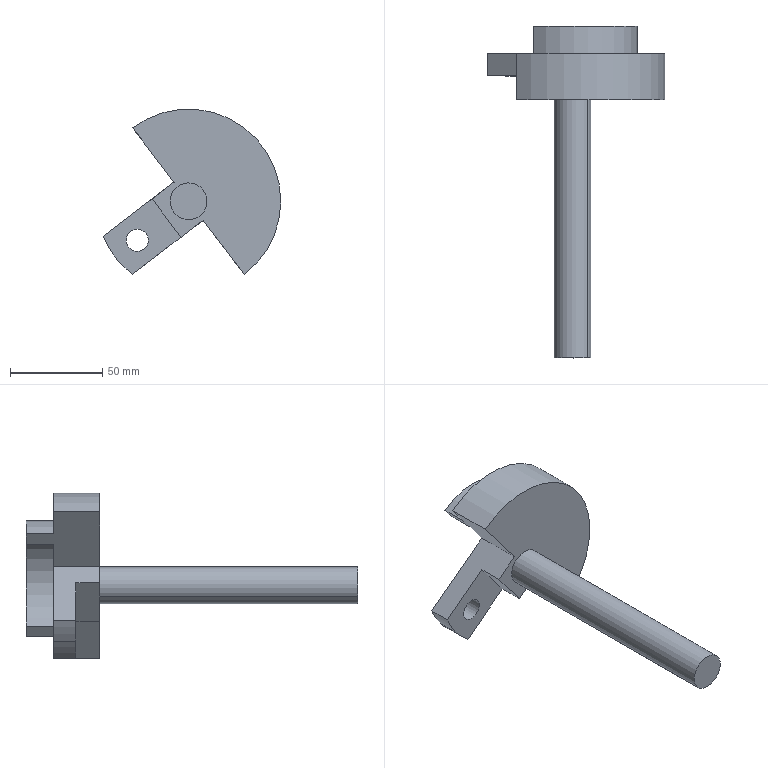Component | SolidWorks | RearRoller-4 | 1 solid | 20 faces | box 96.28 x 180 x 89.77 mm | volume 171683 mm3 | plane 11 | cylinder 9 | commonest cylinder face diameters 100 x3 12 x2 20 x2 56 x1 70 x1
build123d program:
from build123d import *

# Parameters (mm, degrees)
SKETCH2_W      = 83.89
SKETCH2_H      = 46.873
EXTRUDE2_DEPTH = 15
SKETCH3_W      = 56.676
SKETCH3_H      = 55.605
EXTRUDE3_DEPTH = 180.513
SKETCH4_R      = 6
EXTRUDE4_DEPTH = 180.513
SKETCH5_W      = 35
SKETCH5_H      = 13
EXTRUDE5_DEPTH = 148.923


with BuildPart() as part:
    # Sketch1 → Revolve1 (revolve)
    with BuildSketch(Plane.XY, mode=Mode.PRIVATE) as revolve1_sk:
        Polygon((0, 109.146), (28, 109.146), (28, 124.146), (35, 124.146), (35, 109.146), (50, 109.146), (50, 84.146), (10, 84.146), (10, -55.854), (0, -55.854), align=None)
    revolve(revolve1_sk.sketch.rotate(Axis((0, 0, 0), (0, 1, 0)), 90), axis=Axis((0, 0, 0), (0, 1, 0)))

    # Sketch2 → Extrude2 (cut)
    with BuildSketch(Plane(origin=(0, 124.146, 0), x_dir=(1, 0, 0), z_dir=(0, 1, 0))):
        with Locations((-6.945, 23.437)):
            Rectangle(SKETCH2_W, SKETCH2_H)
    extrude(amount=-EXTRUDE2_DEPTH, mode=Mode.SUBTRACT)

    # Sketch3 → Extrude3 (cut, through all)
    with BuildSketch(Plane(origin=(0, 109.146, 0), x_dir=(1, 0, 0), z_dir=(0, 1, 0))):
        with Locations((-41.338, 27.803)):
            Rectangle(SKETCH3_W, SKETCH3_H)
        with Locations((41.338, 27.803)):
            Rectangle(SKETCH3_W, SKETCH3_H)
    extrude(amount=-EXTRUDE3_DEPTH, mode=Mode.SUBTRACT)

    # Sketch4 → Extrude4 (cut, through all)
    with BuildSketch(Plane(origin=(0, 109.146, 0), x_dir=(1, 0, 0), z_dir=(0, 1, 0))):
        with Locations(Location((0, 35, 0), (0, 0, 270))):
            Circle(SKETCH4_R)
    extrude(amount=-EXTRUDE4_DEPTH, mode=Mode.SUBTRACT)

    # Sketch5 → Extrude5 (cut, through all)
    with BuildSketch(Plane(origin=(13, 0, 0), x_dir=(0, 0, -1), z_dir=(1, 0, 0))):
        with Locations((32.5, 90.646)):
            Rectangle(SKETCH5_W, SKETCH5_H)
    extrude(amount=-EXTRUDE5_DEPTH, mode=Mode.SUBTRACT)


solid = part.part

# Placed as in the assembly
solid = solid.moved(Location((-214.784, 404.838, -155), (0, 52.688, 0)))
STEP:
#1=COLOUR_RGB('',0.7922,0.8196,0.9333);
#2=FILL_AREA_STYLE_COLOUR('',#1);
#3=FILL_AREA_STYLE('',(#2));
#4=SURFACE_STYLE_FILL_AREA(#3);
#5=SURFACE_SIDE_STYLE('',(#4));
#6=SURFACE_STYLE_USAGE(.BOTH.,#5);
#7=PRESENTATION_STYLE_ASSIGNMENT((#6));
#8=CARTESIAN_POINT('',(-9.364,19.763,-6.794));
#9=VERTEX_POINT('',#8);
#10=CARTESIAN_POINT('',(-9.74,19.763,-7.081));
#11=VERTEX_POINT('',#10);
#12=CARTESIAN_POINT('',(-9.552,19.763,-6.938));
#13=DIRECTION('',(0.,-1.,-0.));
#14=DIRECTION('',(0.7953,0.,0.6062));
#15=AXIS2_PLACEMENT_3D('',#12,#13,#14);
#16=CIRCLE('',#15,0.2362);
#17=EDGE_CURVE('',#9,#11,#16,.T.);
#18=ORIENTED_EDGE('',*,*,#17,.T.);
#19=CARTESIAN_POINT('',(-9.74,20.236,-7.081));
#20=VERTEX_POINT('',#19);
#21=CARTESIAN_POINT('',(-9.74,13.74,-7.081));
#22=DIRECTION('',(-0.,1.,0.));
#23=VECTOR('',#22,39.37);
#24=LINE('',#21,#23);
#25=EDGE_CURVE('',#11,#20,#24,.T.);
#26=ORIENTED_EDGE('',*,*,#25,.T.);
#27=CARTESIAN_POINT('',(-9.364,20.236,-6.794));
#28=VERTEX_POINT('',#27);
#29=CARTESIAN_POINT('',(-9.552,20.236,-6.938));
#30=DIRECTION('',(-0.,1.,0.));
#31=DIRECTION('',(0.7953,0.,0.6062));
#32=AXIS2_PLACEMENT_3D('',#29,#30,#31);
#33=CIRCLE('',#32,0.2362);
#34=EDGE_CURVE('',#20,#28,#33,.T.);
#35=ORIENTED_EDGE('',*,*,#34,.T.);
#36=CARTESIAN_POINT('',(-9.364,13.74,-6.794));
#37=DIRECTION('',(-0.,1.,0.));
#38=VECTOR('',#37,39.37);
#39=LINE('',#36,#38);
#40=EDGE_CURVE('',#9,#28,#39,.T.);
#41=ORIENTED_EDGE('',*,*,#40,.F.);
#42=EDGE_LOOP('',(#18,#26,#35,#41));
#43=FACE_OUTER_BOUND('',#42,.T.);
#44=CARTESIAN_POINT('',(-9.552,13.74,-6.938));
#45=DIRECTION('',(-0.,1.,0.));
#46=DIRECTION('',(0.7953,0.,0.6062));
#47=AXIS2_PLACEMENT_3D('',#44,#45,#46);
#48=CYLINDRICAL_SURFACE('',#47,0.2362);
#49=ADVANCED_FACE('',(#43),#48,.F.);
#50=CARTESIAN_POINT('',(-8.769,19.251,-6.341));
#51=VERTEX_POINT('',#50);
#52=CARTESIAN_POINT('',(-8.143,19.251,-5.864));
#53=VERTEX_POINT('',#52);
#54=CARTESIAN_POINT('',(-8.456,19.251,-6.102));
#55=DIRECTION('',(0.,-1.,-0.));
#56=DIRECTION('',(-0.7953,0.,-0.6062));
#57=AXIS2_PLACEMENT_3D('',#54,#55,#56);
#58=CIRCLE('',#57,0.3937);
#59=EDGE_CURVE('',#51,#53,#58,.T.);
#60=ORIENTED_EDGE('',*,*,#59,.T.);
#61=CARTESIAN_POINT('',(-8.143,13.74,-5.864));
#62=VERTEX_POINT('',#61);
#63=CARTESIAN_POINT('',(-8.143,15.938,-5.864));
#64=DIRECTION('',(0.,-1.,-0.));
#65=VECTOR('',#64,39.37);
#66=LINE('',#63,#65);
#67=EDGE_CURVE('',#53,#62,#66,.T.);
#68=ORIENTED_EDGE('',*,*,#67,.T.);
#69=CARTESIAN_POINT('',(-8.769,13.74,-6.341));
#70=VERTEX_POINT('',#69);
#71=CARTESIAN_POINT('',(-8.456,13.74,-6.102));
#72=DIRECTION('',(0.,-1.,-0.));
#73=DIRECTION('',(-0.7953,0.,-0.6062));
#74=AXIS2_PLACEMENT_3D('',#71,#72,#73);
#75=CIRCLE('',#74,0.3937);
#76=EDGE_CURVE('',#70,#62,#75,.T.);
#77=ORIENTED_EDGE('',*,*,#76,.F.);
#78=CARTESIAN_POINT('',(-8.769,15.938,-6.341));
#79=DIRECTION('',(0.,-1.,-0.));
#80=VECTOR('',#79,39.37);
#81=LINE('',#78,#80);
#82=EDGE_CURVE('',#51,#70,#81,.T.);
#83=ORIENTED_EDGE('',*,*,#82,.F.);
#84=EDGE_LOOP('',(#60,#68,#77,#83));
#85=FACE_OUTER_BOUND('',#84,.T.);
#86=CARTESIAN_POINT('',(-8.456,15.938,-6.102));
#87=DIRECTION('',(0.,-1.,-0.));
#88=DIRECTION('',(-0.7953,0.,-0.6062));
#89=AXIS2_PLACEMENT_3D('',#86,#87,#88);
#90=CYLINDRICAL_SURFACE('',#89,0.3937);
#91=ADVANCED_FACE('',(#85),#90,.T.);
#92=CARTESIAN_POINT('',(-10.278,20.236,-6.847));
#93=VERTEX_POINT('',#92);
#94=CARTESIAN_POINT('',(-10.022,20.236,-7.296));
#95=VERTEX_POINT('',#94);
#96=CARTESIAN_POINT('',(-8.456,20.236,-6.102));
#97=DIRECTION('',(0.,-1.,-0.));
#98=DIRECTION('',(-0.7953,0.,-0.6062));
#99=AXIS2_PLACEMENT_3D('',#96,#97,#98);
#100=CIRCLE('',#99,1.969);
#101=EDGE_CURVE('',#93,#95,#100,.T.);
#102=ORIENTED_EDGE('',*,*,#101,.T.);
#103=CARTESIAN_POINT('',(-10.022,19.763,-7.296));
#104=VERTEX_POINT('',#103);
#105=CARTESIAN_POINT('',(-10.022,15.938,-7.296));
#106=DIRECTION('',(0.,-1.,-0.));
#107=VECTOR('',#106,39.37);
#108=LINE('',#105,#107);
#109=EDGE_CURVE('',#95,#104,#108,.T.);
#110=ORIENTED_EDGE('',*,*,#109,.T.);
#111=CARTESIAN_POINT('',(-10.278,19.763,-6.847));
#112=VERTEX_POINT('',#111);
#113=CARTESIAN_POINT('',(-8.456,19.763,-6.102));
#114=DIRECTION('',(0.,-1.,-0.));
#115=DIRECTION('',(0.7953,0.,0.6062));
#116=AXIS2_PLACEMENT_3D('',#113,#114,#115);
#117=CIRCLE('',#116,1.969);
#118=EDGE_CURVE('',#112,#104,#117,.T.);
#119=ORIENTED_EDGE('',*,*,#118,.F.);
#120=CARTESIAN_POINT('',(-10.278,15.938,-6.847));
#121=DIRECTION('',(0.,-1.,-0.));
#122=VECTOR('',#121,39.37);
#123=LINE('',#120,#122);
#124=EDGE_CURVE('',#93,#112,#123,.T.);
#125=ORIENTED_EDGE('',*,*,#124,.F.);
#126=EDGE_LOOP('',(#102,#110,#119,#125));
#127=FACE_OUTER_BOUND('',#126,.T.);
#128=CARTESIAN_POINT('',(-8.456,15.938,-6.102));
#129=DIRECTION('',(0.,-1.,-0.));
#130=DIRECTION('',(-0.7953,0.,-0.6062));
#131=AXIS2_PLACEMENT_3D('',#128,#129,#130);
#132=CYLINDRICAL_SURFACE('',#131,1.969);
#133=ADVANCED_FACE('',(#127),#132,.T.);
#134=CARTESIAN_POINT('',(-7.621,20.236,-7.198));
#135=VERTEX_POINT('',#134);
#136=CARTESIAN_POINT('',(-7.263,20.236,-7.668));
#137=VERTEX_POINT('',#136);
#138=CARTESIAN_POINT('',(-6.793,20.236,-8.284));
#139=DIRECTION('',(0.6062,0.,-0.7953));
#140=VECTOR('',#139,39.37);
#141=LINE('',#138,#140);
#142=EDGE_CURVE('',#135,#137,#141,.T.);
#143=ORIENTED_EDGE('',*,*,#142,.F.);
#144=CARTESIAN_POINT('',(-9.291,20.236,-5.006));
#145=VERTEX_POINT('',#144);
#146=CARTESIAN_POINT('',(-8.456,20.236,-6.102));
#147=DIRECTION('',(0.,-1.,-0.));
#148=DIRECTION('',(-0.7953,0.,-0.6062));
#149=AXIS2_PLACEMENT_3D('',#146,#147,#148);
#150=CIRCLE('',#149,1.378);
#151=EDGE_CURVE('',#135,#145,#150,.T.);
#152=ORIENTED_EDGE('',*,*,#151,.T.);
#153=CARTESIAN_POINT('',(-9.649,20.236,-4.537));
#154=VERTEX_POINT('',#153);
#155=CARTESIAN_POINT('',(-10.119,20.236,-3.921));
#156=DIRECTION('',(0.6062,0.,-0.7953));
#157=VECTOR('',#156,39.37);
#158=LINE('',#155,#157);
#159=EDGE_CURVE('',#154,#145,#158,.T.);
#160=ORIENTED_EDGE('',*,*,#159,.F.);
#161=CARTESIAN_POINT('',(-8.456,20.236,-6.102));
#162=DIRECTION('',(0.,-1.,-0.));
#163=DIRECTION('',(-0.7953,0.,-0.6062));
#164=AXIS2_PLACEMENT_3D('',#161,#162,#163);
#165=CIRCLE('',#164,1.969);
#166=EDGE_CURVE('',#137,#154,#165,.T.);
#167=ORIENTED_EDGE('',*,*,#166,.F.);
#168=EDGE_LOOP('',(#143,#152,#160,#167));
#169=FACE_OUTER_BOUND('',#168,.T.);
#170=CARTESIAN_POINT('',(-7.621,20.236,-7.198));
#171=DIRECTION('',(-0.,1.,0.));
#172=DIRECTION('',(0.7953,-0.,0.6062));
#173=AXIS2_PLACEMENT_3D('',#170,#171,#172);
#174=PLANE('',#173);
#175=ADVANCED_FACE('',(#169),#174,.T.);
#176=CARTESIAN_POINT('',(-7.263,19.251,-7.668));
#177=VERTEX_POINT('',#176);
#178=CARTESIAN_POINT('',(-7.263,15.938,-7.668));
#179=DIRECTION('',(0.,-1.,-0.));
#180=VECTOR('',#179,39.37);
#181=LINE('',#178,#180);
#182=EDGE_CURVE('',#137,#177,#181,.T.);
#183=ORIENTED_EDGE('',*,*,#182,.F.);
#184=ORIENTED_EDGE('',*,*,#166,.T.);
#185=CARTESIAN_POINT('',(-9.649,19.251,-4.537));
#186=VERTEX_POINT('',#185);
#187=CARTESIAN_POINT('',(-9.649,15.938,-4.537));
#188=DIRECTION('',(-0.,1.,0.));
#189=VECTOR('',#188,39.37);
#190=LINE('',#187,#189);
#191=EDGE_CURVE('',#186,#154,#190,.T.);
#192=ORIENTED_EDGE('',*,*,#191,.F.);
#193=CARTESIAN_POINT('',(-8.456,19.251,-6.102));
#194=DIRECTION('',(0.,-1.,-0.));
#195=DIRECTION('',(-0.7953,0.,-0.6062));
#196=AXIS2_PLACEMENT_3D('',#193,#194,#195);
#197=CIRCLE('',#196,1.969);
#198=EDGE_CURVE('',#177,#186,#197,.T.);
#199=ORIENTED_EDGE('',*,*,#198,.F.);
#200=EDGE_LOOP('',(#183,#184,#192,#199));
#201=FACE_OUTER_BOUND('',#200,.T.);
#202=CARTESIAN_POINT('',(-8.456,15.938,-6.102));
#203=DIRECTION('',(0.,-1.,-0.));
#204=DIRECTION('',(-0.7953,0.,-0.6062));
#205=AXIS2_PLACEMENT_3D('',#202,#203,#204);
#206=CYLINDRICAL_SURFACE('',#205,1.969);
#207=ADVANCED_FACE('',(#201),#206,.T.);
#208=CARTESIAN_POINT('',(-9.124,20.826,-5.226));
#209=VERTEX_POINT('',#208);
#210=CARTESIAN_POINT('',(-9.124,20.236,-5.226));
#211=VERTEX_POINT('',#210);
#212=CARTESIAN_POINT('',(-9.124,15.938,-5.226));
#213=DIRECTION('',(0.,-1.,-0.));
#214=VECTOR('',#213,39.37);
#215=LINE('',#212,#214);
#216=EDGE_CURVE('',#209,#211,#215,.T.);
#217=ORIENTED_EDGE('',*,*,#216,.F.);
#218=CARTESIAN_POINT('',(-7.788,20.826,-6.979));
#219=VERTEX_POINT('',#218);
#220=CARTESIAN_POINT('',(-8.456,20.826,-6.102));
#221=DIRECTION('',(0.,-1.,-0.));
#222=DIRECTION('',(-0.7953,0.,-0.6062));
#223=AXIS2_PLACEMENT_3D('',#220,#221,#222);
#224=CIRCLE('',#223,1.102);
#225=EDGE_CURVE('',#219,#209,#224,.T.);
#226=ORIENTED_EDGE('',*,*,#225,.F.);
#227=CARTESIAN_POINT('',(-7.788,20.236,-6.979));
#228=VERTEX_POINT('',#227);
#229=CARTESIAN_POINT('',(-7.788,15.938,-6.979));
#230=DIRECTION('',(-0.,1.,0.));
#231=VECTOR('',#230,39.37);
#232=LINE('',#229,#231);
#233=EDGE_CURVE('',#228,#219,#232,.T.);
#234=ORIENTED_EDGE('',*,*,#233,.F.);
#235=CARTESIAN_POINT('',(-8.456,20.236,-6.102));
#236=DIRECTION('',(0.,-1.,-0.));
#237=DIRECTION('',(-0.7953,0.,-0.6062));
#238=AXIS2_PLACEMENT_3D('',#235,#236,#237);
#239=CIRCLE('',#238,1.102);
#240=EDGE_CURVE('',#228,#211,#239,.T.);
#241=ORIENTED_EDGE('',*,*,#240,.T.);
#242=EDGE_LOOP('',(#217,#226,#234,#241));
#243=FACE_OUTER_BOUND('',#242,.T.);
#244=CARTESIAN_POINT('',(-8.456,15.938,-6.102));
#245=DIRECTION('',(0.,-1.,-0.));
#246=DIRECTION('',(-0.7953,0.,-0.6062));
#247=AXIS2_PLACEMENT_3D('',#244,#245,#246);
#248=CYLINDRICAL_SURFACE('',#247,1.102);
#249=ADVANCED_FACE('',(#243),#248,.F.);
#250=CARTESIAN_POINT('',(-9.291,20.826,-5.006));
#251=VERTEX_POINT('',#250);
#252=CARTESIAN_POINT('',(-9.623,20.826,-4.571));
#253=DIRECTION('',(0.6062,0.,-0.7953));
#254=VECTOR('',#253,39.37);
#255=LINE('',#252,#254);
#256=EDGE_CURVE('',#251,#209,#255,.T.);
#257=ORIENTED_EDGE('',*,*,#256,.F.);
#258=CARTESIAN_POINT('',(-7.621,20.826,-7.198));
#259=VERTEX_POINT('',#258);
#260=CARTESIAN_POINT('',(-8.456,20.826,-6.102));
#261=DIRECTION('',(0.,-1.,-0.));
#262=DIRECTION('',(-0.7953,0.,-0.6062));
#263=AXIS2_PLACEMENT_3D('',#260,#261,#262);
#264=CIRCLE('',#263,1.378);
#265=EDGE_CURVE('',#259,#251,#264,.T.);
#266=ORIENTED_EDGE('',*,*,#265,.F.);
#267=CARTESIAN_POINT('',(-9.623,20.826,-4.571));
#268=DIRECTION('',(0.6062,0.,-0.7953));
#269=VECTOR('',#268,39.37);
#270=LINE('',#267,#269);
#271=EDGE_CURVE('',#219,#259,#270,.T.);
#272=ORIENTED_EDGE('',*,*,#271,.F.);
#273=ORIENTED_EDGE('',*,*,#225,.T.);
#274=EDGE_LOOP('',(#257,#266,#272,#273));
#275=FACE_OUTER_BOUND('',#274,.T.);
#276=CARTESIAN_POINT('',(-7.788,20.826,-6.979));
#277=DIRECTION('',(-0.,1.,0.));
#278=DIRECTION('',(0.7953,-0.,0.6062));
#279=AXIS2_PLACEMENT_3D('',#276,#277,#278);
#280=PLANE('',#279);
#281=ADVANCED_FACE('',(#275),#280,.T.);
#282=CARTESIAN_POINT('',(-9.291,15.938,-5.006));
#283=DIRECTION('',(-0.,1.,0.));
#284=VECTOR('',#283,39.37);
#285=LINE('',#282,#284);
#286=EDGE_CURVE('',#145,#251,#285,.T.);
#287=ORIENTED_EDGE('',*,*,#286,.F.);
#288=ORIENTED_EDGE('',*,*,#151,.F.);
#289=CARTESIAN_POINT('',(-7.621,16.452,-7.198));
#290=DIRECTION('',(-0.,1.,0.));
#291=VECTOR('',#290,39.37);
#292=LINE('',#289,#291);
#293=EDGE_CURVE('',#135,#259,#292,.T.);
#294=ORIENTED_EDGE('',*,*,#293,.T.);
#295=ORIENTED_EDGE('',*,*,#265,.T.);
#296=EDGE_LOOP('',(#287,#288,#294,#295));
#297=FACE_OUTER_BOUND('',#296,.T.);
#298=CARTESIAN_POINT('',(-8.456,15.938,-6.102));
#299=DIRECTION('',(0.,-1.,-0.));
#300=DIRECTION('',(-0.7953,0.,-0.6062));
#301=AXIS2_PLACEMENT_3D('',#298,#299,#300);
#302=CYLINDRICAL_SURFACE('',#301,1.378);
#303=ADVANCED_FACE('',(#297),#302,.T.);
#304=CARTESIAN_POINT('',(-9.552,20.236,-6.938));
#305=DIRECTION('',(-0.,1.,0.));
#306=DIRECTION('',(0.7953,0.,0.6062));
#307=AXIS2_PLACEMENT_3D('',#304,#305,#306);
#308=CIRCLE('',#307,0.2362);
#309=EDGE_CURVE('',#28,#20,#308,.T.);
#310=ORIENTED_EDGE('',*,*,#309,.F.);
#311=ORIENTED_EDGE('',*,*,#34,.F.);
#312=EDGE_LOOP('',(#310,#311));
#313=FACE_BOUND('',#312,.T.);
#314=CARTESIAN_POINT('',(-8.146,20.236,-6.509));
#315=VERTEX_POINT('',#314);
#316=CARTESIAN_POINT('',(-6.793,20.236,-8.284));
#317=DIRECTION('',(0.6062,0.,-0.7953));
#318=VECTOR('',#317,39.37);
#319=LINE('',#316,#318);
#320=EDGE_CURVE('',#315,#228,#319,.T.);
#321=ORIENTED_EDGE('',*,*,#320,.F.);
#322=CARTESIAN_POINT('',(-9.658,20.236,-7.662));
#323=VERTEX_POINT('',#322);
#324=CARTESIAN_POINT('',(-9.887,20.236,-7.836));
#325=DIRECTION('',(0.7953,-0.,0.6062));
#326=VECTOR('',#325,39.37);
#327=LINE('',#324,#326);
#328=EDGE_CURVE('',#323,#315,#327,.T.);
#329=ORIENTED_EDGE('',*,*,#328,.F.);
#330=CARTESIAN_POINT('',(-8.456,20.236,-6.102));
#331=DIRECTION('',(0.,-1.,-0.));
#332=DIRECTION('',(-0.7953,0.,-0.6062));
#333=AXIS2_PLACEMENT_3D('',#330,#331,#332);
#334=CIRCLE('',#333,1.969);
#335=EDGE_CURVE('',#95,#323,#334,.T.);
#336=ORIENTED_EDGE('',*,*,#335,.F.);
#337=ORIENTED_EDGE('',*,*,#101,.F.);
#338=CARTESIAN_POINT('',(-8.766,20.236,-5.695));
#339=VERTEX_POINT('',#338);
#340=CARTESIAN_POINT('',(-10.507,20.236,-7.022));
#341=DIRECTION('',(-0.7953,0.,-0.6062));
#342=VECTOR('',#341,39.37);
#343=LINE('',#340,#342);
#344=EDGE_CURVE('',#339,#93,#343,.T.);
#345=ORIENTED_EDGE('',*,*,#344,.F.);
#346=CARTESIAN_POINT('',(-10.119,20.236,-3.921));
#347=DIRECTION('',(0.6062,0.,-0.7953));
#348=VECTOR('',#347,39.37);
#349=LINE('',#346,#348);
#350=EDGE_CURVE('',#211,#339,#349,.T.);
#351=ORIENTED_EDGE('',*,*,#350,.F.);
#352=ORIENTED_EDGE('',*,*,#240,.F.);
#353=EDGE_LOOP('',(#321,#329,#336,#337,#345,#351,#352));
#354=FACE_OUTER_BOUND('',#353,.T.);
#355=CARTESIAN_POINT('',(-7.621,20.236,-7.198));
#356=DIRECTION('',(-0.,1.,0.));
#357=DIRECTION('',(0.7953,-0.,0.6062));
#358=AXIS2_PLACEMENT_3D('',#355,#356,#357);
#359=PLANE('',#358);
#360=ADVANCED_FACE('',(#313,#354),#359,.T.);
#361=ORIENTED_EDGE('',*,*,#109,.F.);
#362=ORIENTED_EDGE('',*,*,#335,.T.);
#363=CARTESIAN_POINT('',(-9.658,19.763,-7.662));
#364=VERTEX_POINT('',#363);
#365=CARTESIAN_POINT('',(-9.658,15.938,-7.662));
#366=DIRECTION('',(-0.,1.,0.));
#367=VECTOR('',#366,39.37);
#368=LINE('',#365,#367);
#369=EDGE_CURVE('',#364,#323,#368,.T.);
#370=ORIENTED_EDGE('',*,*,#369,.F.);
#371=CARTESIAN_POINT('',(-8.456,19.763,-6.102));
#372=DIRECTION('',(0.,-1.,-0.));
#373=DIRECTION('',(0.7953,0.,0.6062));
#374=AXIS2_PLACEMENT_3D('',#371,#372,#373);
#375=CIRCLE('',#374,1.969);
#376=EDGE_CURVE('',#104,#364,#375,.T.);
#377=ORIENTED_EDGE('',*,*,#376,.F.);
#378=EDGE_LOOP('',(#361,#362,#370,#377));
#379=FACE_OUTER_BOUND('',#378,.T.);
#380=CARTESIAN_POINT('',(-8.456,15.938,-6.102));
#381=DIRECTION('',(0.,-1.,-0.));
#382=DIRECTION('',(-0.7953,0.,-0.6062));
#383=AXIS2_PLACEMENT_3D('',#380,#381,#382);
#384=CYLINDRICAL_SURFACE('',#383,1.969);
#385=ADVANCED_FACE('',(#379),#384,.T.);
#386=CARTESIAN_POINT('',(-9.236,19.251,-6.053));
#387=VERTEX_POINT('',#386);
#388=CARTESIAN_POINT('',(-8.616,19.251,-6.867));
#389=VERTEX_POINT('',#388);
#390=CARTESIAN_POINT('',(-10.119,19.251,-4.895));
#391=DIRECTION('',(0.6062,0.,-0.7953));
#392=VECTOR('',#391,39.37);
#393=LINE('',#390,#392);
#394=EDGE_CURVE('',#387,#389,#393,.T.);
#395=ORIENTED_EDGE('',*,*,#394,.T.);
#396=CARTESIAN_POINT('',(-8.146,19.251,-6.509));
#397=VERTEX_POINT('',#396);
#398=CARTESIAN_POINT('',(-8.146,19.251,-6.509));
#399=DIRECTION('',(-0.7953,0.,-0.6062));
#400=VECTOR('',#399,39.37);
#401=LINE('',#398,#400);
#402=EDGE_CURVE('',#397,#389,#401,.T.);
#403=ORIENTED_EDGE('',*,*,#402,.F.);
#404=CARTESIAN_POINT('',(-7.263,19.251,-7.668));
#405=DIRECTION('',(-0.6062,-0.,0.7953));
#406=VECTOR('',#405,39.37);
#407=LINE('',#404,#406);
#408=EDGE_CURVE('',#177,#397,#407,.T.);
#409=ORIENTED_EDGE('',*,*,#408,.F.);
#410=ORIENTED_EDGE('',*,*,#198,.T.);
#411=CARTESIAN_POINT('',(-8.766,19.251,-5.695));
#412=VERTEX_POINT('',#411);
#413=CARTESIAN_POINT('',(-7.263,19.251,-7.668));
#414=DIRECTION('',(-0.6062,-0.,0.7953));
#415=VECTOR('',#414,39.37);
#416=LINE('',#413,#415);
#417=EDGE_CURVE('',#412,#186,#416,.T.);
#418=ORIENTED_EDGE('',*,*,#417,.F.);
#419=CARTESIAN_POINT('',(-8.766,19.251,-5.695));
#420=DIRECTION('',(0.7953,-0.,0.6062));
#421=VECTOR('',#420,39.37);
#422=LINE('',#419,#421);
#423=EDGE_CURVE('',#387,#412,#422,.T.);
#424=ORIENTED_EDGE('',*,*,#423,.F.);
#425=EDGE_LOOP('',(#395,#403,#409,#410,#418,#424));
#426=FACE_OUTER_BOUND('',#425,.T.);
#427=ORIENTED_EDGE('',*,*,#59,.F.);
#428=CARTESIAN_POINT('',(-8.456,19.251,-6.102));
#429=DIRECTION('',(0.,-1.,-0.));
#430=DIRECTION('',(-0.7953,0.,-0.6062));
#431=AXIS2_PLACEMENT_3D('',#428,#429,#430);
#432=CIRCLE('',#431,0.3937);
#433=EDGE_CURVE('',#53,#51,#432,.T.);
#434=ORIENTED_EDGE('',*,*,#433,.F.);
#435=EDGE_LOOP('',(#427,#434));
#436=FACE_BOUND('',#435,.T.);
#437=CARTESIAN_POINT('',(-7.263,19.251,-7.668));
#438=DIRECTION('',(0.,-1.,-0.));
#439=DIRECTION('',(-0.7953,0.,-0.6062));
#440=AXIS2_PLACEMENT_3D('',#437,#438,#439);
#441=PLANE('',#440);
#442=ADVANCED_FACE('',(#426,#436),#441,.T.);
#443=ORIENTED_EDGE('',*,*,#67,.F.);
#444=ORIENTED_EDGE('',*,*,#433,.T.);
#445=ORIENTED_EDGE('',*,*,#82,.T.);
#446=CARTESIAN_POINT('',(-8.456,13.74,-6.102));
#447=DIRECTION('',(0.,-1.,-0.));
#448=DIRECTION('',(-0.7953,0.,-0.6062));
#449=AXIS2_PLACEMENT_3D('',#446,#447,#448);
#450=CIRCLE('',#449,0.3937);
#451=EDGE_CURVE('',#62,#70,#450,.T.);
#452=ORIENTED_EDGE('',*,*,#451,.F.);
#453=EDGE_LOOP('',(#443,#444,#445,#452));
#454=FACE_OUTER_BOUND('',#453,.T.);
#455=CARTESIAN_POINT('',(-8.456,15.938,-6.102));
#456=DIRECTION('',(0.,-1.,-0.));
#457=DIRECTION('',(-0.7953,0.,-0.6062));
#458=AXIS2_PLACEMENT_3D('',#455,#456,#457);
#459=CYLINDRICAL_SURFACE('',#458,0.3937);
#460=ADVANCED_FACE('',(#454),#459,.T.);
#461=ORIENTED_EDGE('',*,*,#76,.T.);
#462=ORIENTED_EDGE('',*,*,#451,.T.);
#463=EDGE_LOOP('',(#461,#462));
#464=FACE_OUTER_BOUND('',#463,.T.);
#465=CARTESIAN_POINT('',(-8.217,13.74,-6.415));
#466=DIRECTION('',(0.,-1.,-0.));
#467=DIRECTION('',(-0.7953,0.,-0.6062));
#468=AXIS2_PLACEMENT_3D('',#465,#466,#467);
#469=PLANE('',#468);
#470=ADVANCED_FACE('',(#464),#469,.T.);
#471=ORIENTED_EDGE('',*,*,#216,.T.);
#472=ORIENTED_EDGE('',*,*,#350,.T.);
#473=CARTESIAN_POINT('',(-8.766,13.74,-5.695));
#474=DIRECTION('',(-0.,1.,0.));
#475=VECTOR('',#474,39.37);
#476=LINE('',#473,#475);
#477=EDGE_CURVE('',#412,#339,#476,.T.);
#478=ORIENTED_EDGE('',*,*,#477,.F.);
#479=ORIENTED_EDGE('',*,*,#417,.T.);
#480=ORIENTED_EDGE('',*,*,#191,.T.);
#481=ORIENTED_EDGE('',*,*,#159,.T.);
#482=ORIENTED_EDGE('',*,*,#286,.T.);
#483=ORIENTED_EDGE('',*,*,#256,.T.);
#484=EDGE_LOOP('',(#471,#472,#478,#479,#480,#481,#482,#483));
#485=FACE_OUTER_BOUND('',#484,.T.);
#486=CARTESIAN_POINT('',(-9.623,16.452,-4.571));
#487=DIRECTION('',(0.7953,-0.,0.6062));
#488=DIRECTION('',(0.6062,0.,-0.7953));
#489=AXIS2_PLACEMENT_3D('',#486,#487,#488);
#490=PLANE('',#489);
#491=ADVANCED_FACE('',(#485),#490,.F.);
#492=ORIENTED_EDGE('',*,*,#233,.T.);
#493=ORIENTED_EDGE('',*,*,#271,.T.);
#494=ORIENTED_EDGE('',*,*,#293,.F.);
#495=ORIENTED_EDGE('',*,*,#142,.T.);
#496=ORIENTED_EDGE('',*,*,#182,.T.);
#497=ORIENTED_EDGE('',*,*,#408,.T.);
#498=CARTESIAN_POINT('',(-8.146,13.74,-6.509));
#499=DIRECTION('',(-0.,1.,0.));
#500=VECTOR('',#499,39.37);
#501=LINE('',#498,#500);
#502=EDGE_CURVE('',#397,#315,#501,.T.);
#503=ORIENTED_EDGE('',*,*,#502,.T.);
#504=ORIENTED_EDGE('',*,*,#320,.T.);
#505=EDGE_LOOP('',(#492,#493,#494,#495,#496,#497,#503,#504));
#506=FACE_OUTER_BOUND('',#505,.T.);
#507=CARTESIAN_POINT('',(-9.623,16.452,-4.571));
#508=DIRECTION('',(0.7953,-0.,0.6062));
#509=DIRECTION('',(0.6062,0.,-0.7953));
#510=AXIS2_PLACEMENT_3D('',#507,#508,#509);
#511=PLANE('',#510);
#512=ADVANCED_FACE('',(#506),#511,.F.);
#513=CARTESIAN_POINT('',(-9.236,19.763,-6.053));
#514=VERTEX_POINT('',#513);
#515=CARTESIAN_POINT('',(-10.507,19.763,-7.022));
#516=DIRECTION('',(0.7953,-0.,0.6062));
#517=VECTOR('',#516,39.37);
#518=LINE('',#515,#517);
#519=EDGE_CURVE('',#112,#514,#518,.T.);
#520=ORIENTED_EDGE('',*,*,#519,.T.);
#521=CARTESIAN_POINT('',(-9.236,13.74,-6.053));
#522=DIRECTION('',(0.,-1.,-0.));
#523=VECTOR('',#522,39.37);
#524=LINE('',#521,#523);
#525=EDGE_CURVE('',#514,#387,#524,.T.);
#526=ORIENTED_EDGE('',*,*,#525,.T.);
#527=ORIENTED_EDGE('',*,*,#423,.T.);
#528=ORIENTED_EDGE('',*,*,#477,.T.);
#529=ORIENTED_EDGE('',*,*,#344,.T.);
#530=ORIENTED_EDGE('',*,*,#124,.T.);
#531=EDGE_LOOP('',(#520,#526,#527,#528,#529,#530));
#532=FACE_OUTER_BOUND('',#531,.T.);
#533=CARTESIAN_POINT('',(-10.507,13.74,-7.022));
#534=DIRECTION('',(0.6062,0.,-0.7953));
#535=DIRECTION('',(-0.7953,0.,-0.6062));
#536=AXIS2_PLACEMENT_3D('',#533,#534,#535);
#537=PLANE('',#536);
#538=ADVANCED_FACE('',(#532),#537,.F.);
#539=ORIENTED_EDGE('',*,*,#402,.T.);
#540=CARTESIAN_POINT('',(-8.616,19.763,-6.867));
#541=VERTEX_POINT('',#540);
#542=CARTESIAN_POINT('',(-8.616,19.251,-6.867));
#543=DIRECTION('',(0.,-1.,-0.));
#544=VECTOR('',#543,39.37);
#545=LINE('',#542,#544);
#546=EDGE_CURVE('',#541,#389,#545,.T.);
#547=ORIENTED_EDGE('',*,*,#546,.F.);
#548=CARTESIAN_POINT('',(-9.711,19.763,-7.703));
#549=DIRECTION('',(0.7953,-0.,0.6062));
#550=VECTOR('',#549,39.37);
#551=LINE('',#548,#550);
#552=EDGE_CURVE('',#364,#541,#551,.T.);
#553=ORIENTED_EDGE('',*,*,#552,.F.);
#554=ORIENTED_EDGE('',*,*,#369,.T.);
#555=ORIENTED_EDGE('',*,*,#328,.T.);
#556=ORIENTED_EDGE('',*,*,#502,.F.);
#557=EDGE_LOOP('',(#539,#547,#553,#554,#555,#556));
#558=FACE_OUTER_BOUND('',#557,.T.);
#559=CARTESIAN_POINT('',(-9.887,13.74,-7.836));
#560=DIRECTION('',(-0.6062,-0.,0.7953));
#561=DIRECTION('',(0.7953,-0.,0.6062));
#562=AXIS2_PLACEMENT_3D('',#559,#560,#561);
#563=PLANE('',#562);
#564=ADVANCED_FACE('',(#558),#563,.F.);
#565=ORIENTED_EDGE('',*,*,#25,.F.);
#566=CARTESIAN_POINT('',(-9.552,19.763,-6.938));
#567=DIRECTION('',(0.,-1.,-0.));
#568=DIRECTION('',(0.7953,0.,0.6062));
#569=AXIS2_PLACEMENT_3D('',#566,#567,#568);
#570=CIRCLE('',#569,0.2362);
#571=EDGE_CURVE('',#11,#9,#570,.T.);
#572=ORIENTED_EDGE('',*,*,#571,.T.);
#573=ORIENTED_EDGE('',*,*,#40,.T.);
#574=ORIENTED_EDGE('',*,*,#309,.T.);
#575=EDGE_LOOP('',(#565,#572,#573,#574));
#576=FACE_OUTER_BOUND('',#575,.T.);
#577=CARTESIAN_POINT('',(-9.552,13.74,-6.938));
#578=DIRECTION('',(-0.,1.,0.));
#579=DIRECTION('',(0.7953,0.,0.6062));
#580=AXIS2_PLACEMENT_3D('',#577,#578,#579);
#581=CYLINDRICAL_SURFACE('',#580,0.2362);
#582=ADVANCED_FACE('',(#576),#581,.F.);
#583=CARTESIAN_POINT('',(-10.119,19.763,-4.895));
#584=DIRECTION('',(0.6062,0.,-0.7953));
#585=VECTOR('',#584,39.37);
#586=LINE('',#583,#585);
#587=EDGE_CURVE('',#514,#541,#586,.T.);
#588=ORIENTED_EDGE('',*,*,#587,.T.);
#589=ORIENTED_EDGE('',*,*,#546,.T.);
#590=ORIENTED_EDGE('',*,*,#394,.F.);
#591=ORIENTED_EDGE('',*,*,#525,.F.);
#592=EDGE_LOOP('',(#588,#589,#590,#591));
#593=FACE_OUTER_BOUND('',#592,.T.);
#594=CARTESIAN_POINT('',(-10.119,19.251,-4.895));
#595=DIRECTION('',(0.7953,-0.,0.6062));
#596=DIRECTION('',(0.6062,0.,-0.7953));
#597=AXIS2_PLACEMENT_3D('',#594,#595,#596);
#598=PLANE('',#597);
#599=ADVANCED_FACE('',(#593),#598,.F.);
#600=ORIENTED_EDGE('',*,*,#118,.T.);
#601=ORIENTED_EDGE('',*,*,#376,.T.);
#602=ORIENTED_EDGE('',*,*,#552,.T.);
#603=ORIENTED_EDGE('',*,*,#587,.F.);
#604=ORIENTED_EDGE('',*,*,#519,.F.);
#605=EDGE_LOOP('',(#600,#601,#602,#603,#604));
#606=FACE_OUTER_BOUND('',#605,.T.);
#607=ORIENTED_EDGE('',*,*,#17,.F.);
#608=ORIENTED_EDGE('',*,*,#571,.F.);
#609=EDGE_LOOP('',(#607,#608));
#610=FACE_BOUND('',#609,.T.);
#611=CARTESIAN_POINT('',(-11.215,19.763,-5.73));
#612=DIRECTION('',(-0.,1.,0.));
#613=DIRECTION('',(0.7953,-0.,0.6062));
#614=AXIS2_PLACEMENT_3D('',#611,#612,#613);
#615=PLANE('',#614);
#616=ADVANCED_FACE('',(#606,#610),#615,.F.);
#617=CLOSED_SHELL('',(#49,#91,#133,#175,#207,#249,#281,#303,#360,#385,#442,#460,#470,#491,#512,#538,#564,#582,#599,#616));
#618=MANIFOLD_SOLID_BREP('',#617);
#619=STYLED_ITEM('',(#7),#618);
#620=PRESENTATION_LAYER_ASSIGNMENT('','',(#619));
#621=CARTESIAN_POINT('',(0.,0.,0.));
#622=DIRECTION('',(0.,0.,1.));
#623=DIRECTION('',(1.,0.,0.));
#624=AXIS2_PLACEMENT_3D('',#621,#622,#623);
#625=(LENGTH_UNIT()NAMED_UNIT(*)SI_UNIT($,.METRE.));
#626=LENGTH_MEASURE_WITH_UNIT(LENGTH_MEASURE(0.0254),#625);
#627=DIMENSIONAL_EXPONENTS(1.,0.,0.,0.,0.,0.,0.);
#628=(CONVERSION_BASED_UNIT('',#626)LENGTH_UNIT()NAMED_UNIT(#627));
#629=UNCERTAINTY_MEASURE_WITH_UNIT(LENGTH_MEASURE(0.00001),#628,'','');
#630=(NAMED_UNIT(*)PLANE_ANGLE_UNIT()SI_UNIT($,.RADIAN.));
#631=(NAMED_UNIT(*)SI_UNIT($,.STERADIAN.)SOLID_ANGLE_UNIT());
#632=(GEOMETRIC_REPRESENTATION_CONTEXT(3)GLOBAL_UNCERTAINTY_ASSIGNED_CONTEXT((#629))GLOBAL_UNIT_ASSIGNED_CONTEXT((#628,#630,#631))REPRESENTATION_CONTEXT('',''));
#633=ADVANCED_BREP_SHAPE_REPRESENTATION('',(#618,#624),#632);
#634=(LENGTH_UNIT()NAMED_UNIT(*)SI_UNIT($,.METRE.));
#635=LENGTH_MEASURE_WITH_UNIT(LENGTH_MEASURE(0.0254),#634);
#636=DIMENSIONAL_EXPONENTS(1.,0.,0.,0.,0.,0.,0.);
#637=(CONVERSION_BASED_UNIT('',#635)LENGTH_UNIT()NAMED_UNIT(#636));
#638=UNCERTAINTY_MEASURE_WITH_UNIT(LENGTH_MEASURE(0.00001),#637,'','');
#639=(NAMED_UNIT(*)PLANE_ANGLE_UNIT()SI_UNIT($,.RADIAN.));
#640=(NAMED_UNIT(*)SI_UNIT($,.STERADIAN.)SOLID_ANGLE_UNIT());
#641=(GEOMETRIC_REPRESENTATION_CONTEXT(3)GLOBAL_UNCERTAINTY_ASSIGNED_CONTEXT((#638))GLOBAL_UNIT_ASSIGNED_CONTEXT((#637,#639,#640))REPRESENTATION_CONTEXT('',''));
#642=MECHANICAL_DESIGN_GEOMETRIC_PRESENTATION_REPRESENTATION('',(#619),#641);